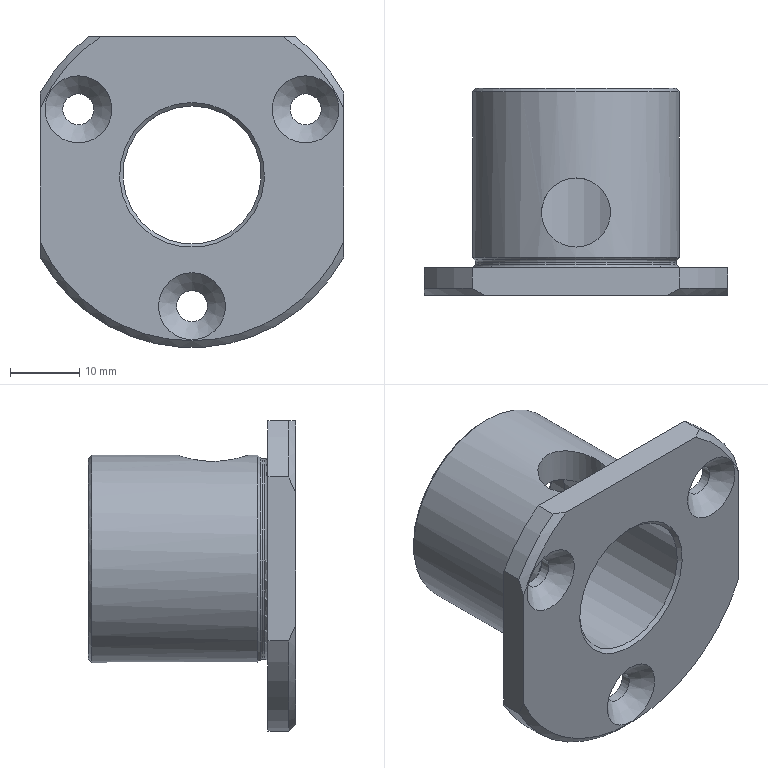Component | NX | GENEVA_SLEEVE | 1 solid | 31 faces | volume 13543 mm3 | cylinder 11 | cone 11 | plane 7 | torus 2 | commonest cylinder face diameters 50 x3 4.5 x3 30 x1 20 x1 29 x1 27 x1 10 x1